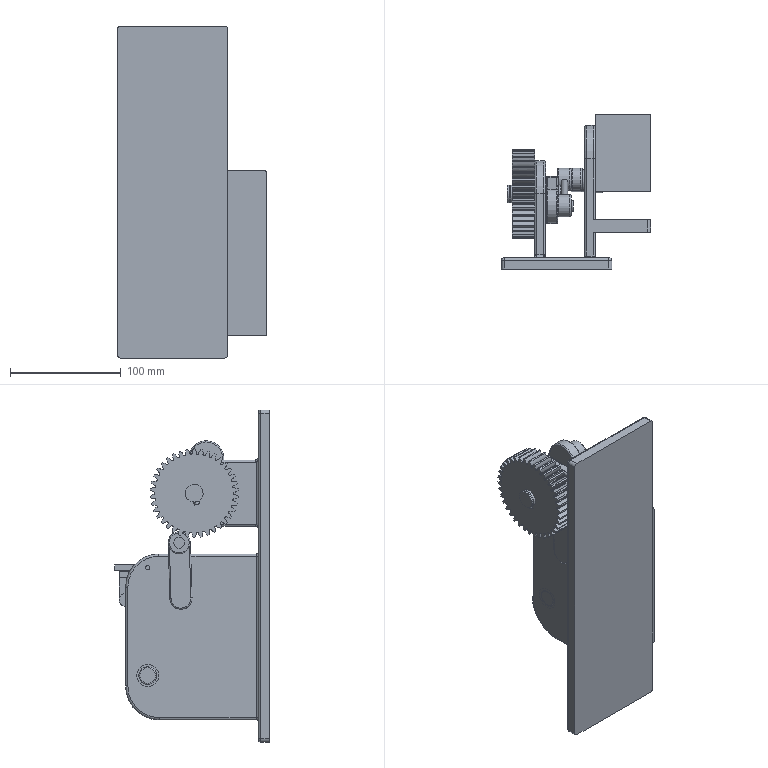Assembly | NX | mm | 15 component files | 17 solids | 487 faces | box 135 x 140 x 300 mm | volume 787858 mm3 | other 190 | cylinder 142 | plane 110 | torus 37 | spline 8 | commonest cylinder face diameters 71 x38 4 x26 16 x12 20 x12 5 x10 6 x10 2 x8 0.4 x6
Bill of materials:
unnamed part 1 | 1 |  | Thin-walled plain cylindrical ring or tube with a concentric through-bore and flat ends.
unnamed part 2 | 1 |  | Short solid block with an obround (stadium-shaped) outline: flat top and bottom faces, semicircular ends, and slightly rounded or chamfered top and bottom edges.
unnamed part 3 | 1 |  | Long solid bar with an obround (stadium-shaped) outline: flat top and bottom faces, semicircular ends, and small edge rounds.
unnamed part 4 | 1 |  | Cylindrical pin with a raised collar band offset from the middle, one radial through-hole across the shaft on the longer side of the collar, and chamfered or rounded ends.
unnamed part 5 | 1 |  | Flat obround arm plate. One end has a cylindrical pin sticking out of one face. The other end has a bore with a keyway notch, surrounded by a slightly raised circular boss on the opposite face.
unnamed part 6 | 1 |  | Thin-walled plain cylindrical ring or tube with a concentric through-bore and flat ends.
unnamed part 7 | 1 |  | Thin-walled plain cylindrical ring or tube with a concentric through-bore and flat ends.
unnamed part 8 | 1 |  | Straight-tooth spur gear: a flat disc with many external teeth and a central circular bore with one keyway notch.
unnamed part 9 | 1 |  | Obround crank arm. One end has a cylindrical pin on one face. The other end has, on the opposite face, a stepped cylindrical boss (thin shoulder plus a larger cylinder) ending in a small square-section projection.
unnamed part 10 | 1 |  | Connecting link made of two cylindrical eye rings, each with a through-hole, joined by a slender straight round rod.
unnamed part 11 | 1 |  | Flat rectangular plate with two short cylindrical pins sticking out from one edge, parallel to the plate plane.
unnamed part 12 | 1 |  | Flat square or rectangular plate with a long slender round rod running perpendicular from its underside, plus a tab hanging down from one edge with a rounded end and a small through-hole.
unnamed part 13 | 1 |  | Flat lever/crank-style arm: a straight bar of constant thickness with a circular enlarged end containing a square through-hole, and a rounded opposite end carrying a short solid cylindrical pin projecting perpendicular to one face.
unnamed part 14 | 1 |  | Solid cylindrical pin with plain flat ends and a narrow circumferential groove near each end; one side view shows two shallow light-colored elongated features along one side.
unnamed part 15 | 1 |  | Bracket made of a rectangular base plate with two parallel lug plates standing perpendicular to it. The shorter lug has a rounded end with one round hole. The taller, wider lug has two larger round holes, two very small holes, and a rounded corner, plus a flat flange bent or extended at a right angle from its side.
Mates:
1. fix | Base 1 component
2. touch align | Cylindrical_Gear_38x2 1 face | Shaft 1 face
3. distance | Cylindrical_Gear_38x2 1 face | Shaft 1 face
4. distance | Crank 1 face | Shaft 1 face
5. touch align | Crank 1 face | Shaft 1 face
6. distance | Crank 1 face | Base 1 face
7. touch align | Connecting_Rod 1 face | Crank 1 face
8. distance | Connecting_Rod 1 face | Crank 1 face
9. touch align | Connecting_Rod 1 face | Rocker 1 face
10. touch align | Rocker 1 face | Rocker_Connecting_Rod 1 face
11. touch align | Print_Block 1 face | Rocker_Connecting_Rod 1 face
12. touch align | Guide_Block 1 face | Bushing 1 face
13. touch align | Print_Block 1 face | Guide_Block 1 face
14. distance | Rocker_Connecting_Rod 1 face | Print_Block 1 face
15. distance | Rocker_Connecting_Rod 1 face | Base 1 face